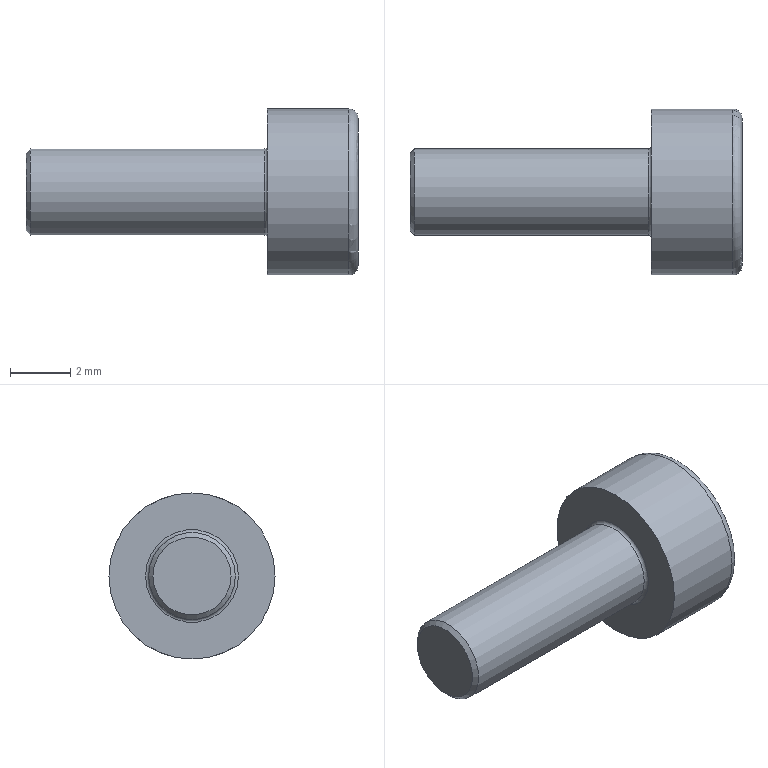Component | NX | GB-T70_1-2000_M3X8_2 | 1 solid | 27 faces | volume 112 mm3 | plane 15 | cone 8 | cylinder 2 | torus 2 | commonest cylinder face diameters 2.874 x1 5.5 x1